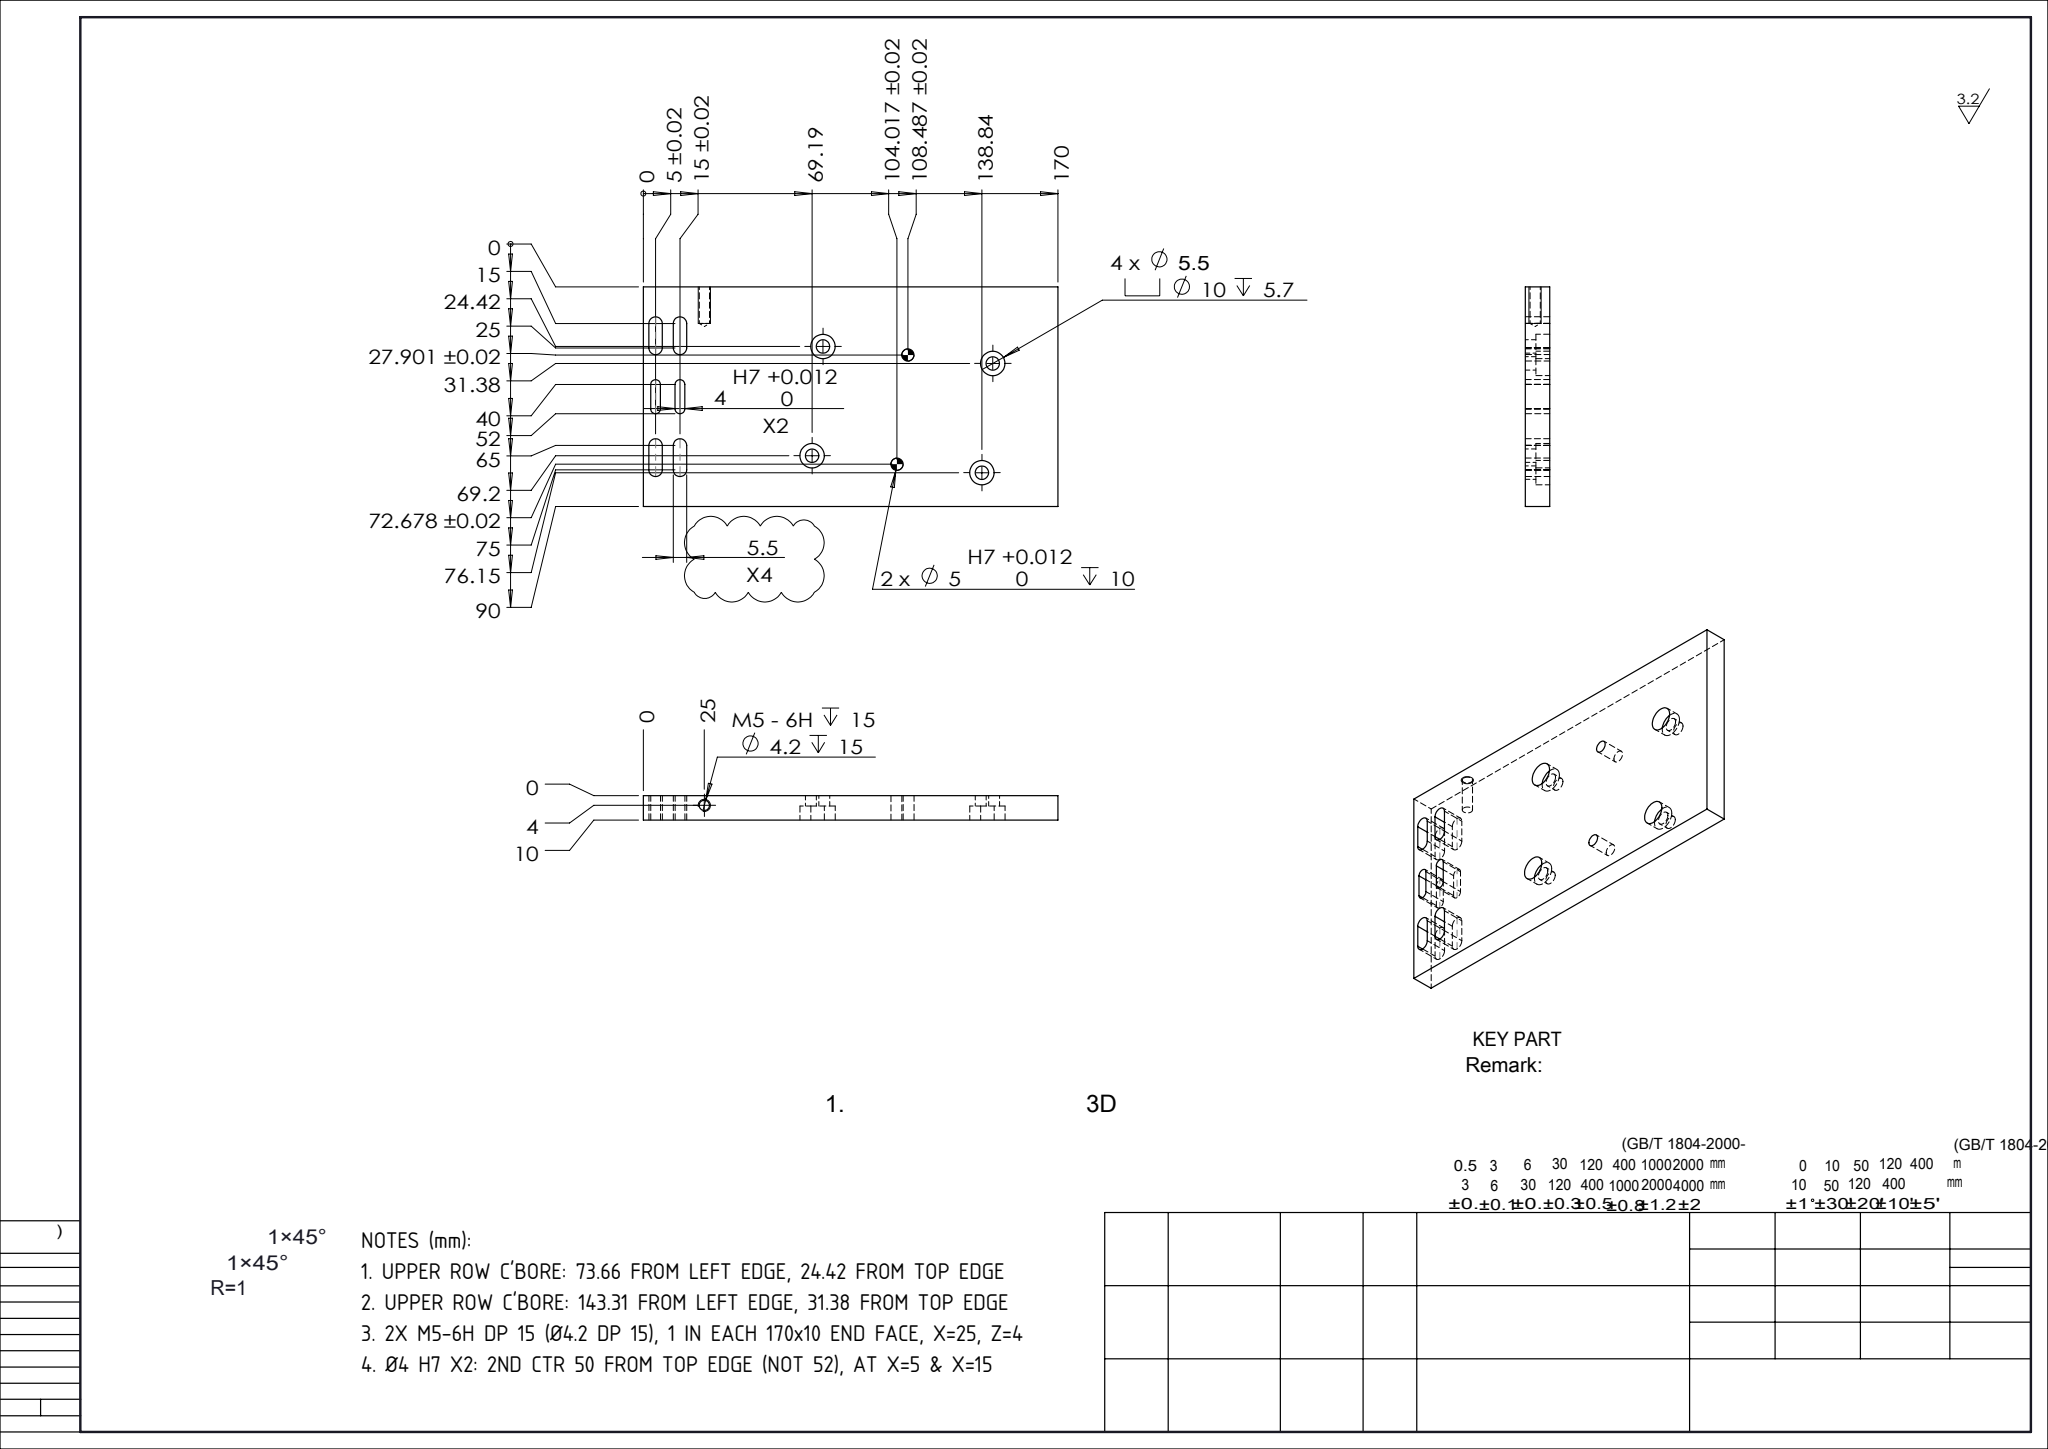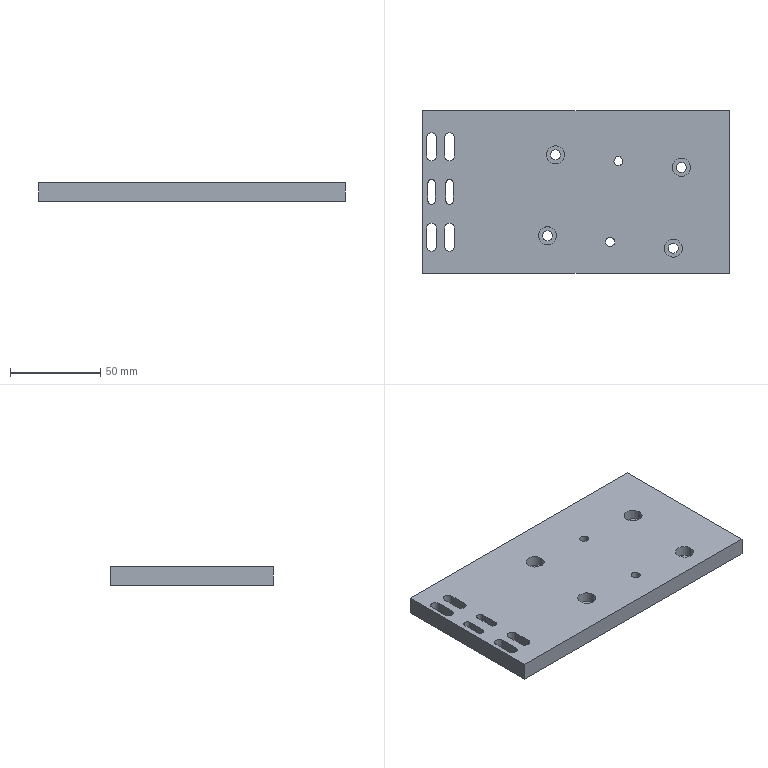Part | SolidWorks | mm | 1 solid | 58 faces | box 170 x 90 x 10 mm | volume 145993 mm3 | cylinder 34 | plane 22 | cone 2 | commonest cylinder face diameters 5.5 x16 10 x8 5 x4 4 x4 4.2 x2
Drawing notes:
UPPER ROW C'BORE: 73.66 FROM LEFT EDGE, 24.42 FROM TOP EDGE | from the solid: Ø5.5 thru w/ Ø10↧5.7 c'bore at x=73.66, y=65.58 (=90-24.42)
UPPER ROW C'BORE: 143.31 FROM LEFT EDGE, 31.38 FROM TOP EDGE | from the solid: Ø5.5 thru w/ Ø10↧5.7 c'bore at x=143.31, y=58.62 (=90-31.38)
2X M5-6H DP 15 (Ø4.2 DP 15), 1 IN EACH 170x10 END FACE, X=25, Z=4 | from the solid: [4.2,'y',[25.0,null,4.0],15.0,2] - two Ø4.2 y-axis holes in y=0 and y=90 faces
Ø4 H7 X2: 2ND CTR 50 FROM TOP EDGE (NOT 52), AT X=5 & X=15 | from the solid: cylinders Ø4 z-axis at [5,50],[15,50] and [5,40],[15,40]; bbox Y=90 so 40 & 50 from top edge
build123d program:
from build123d import *

# Parameters (mm, degrees)
SKETCH1_W                  = 170
SKETCH1_H                  = 90
BOSS_EXTRUDE1_DEPTH        = 10
CUT_EXTRUDE1_DEPTH         = 10
LPATTERN1_COUNT            = 2
LPATTERN1_PITCH            = 50
LPATTERN1_COUNT_DIR2       = 2
LPATTERN1_PITCH_DIR2       = 10
CUT_EXTRUDE2_DEPTH         = 10
HOLE_WIZARD_K_D            = 5.5
HOLE_WIZARD_K_CBORE_D      = 10
HOLE_WIZARD_K_CBORE_DEPTH  = 5.7
SIZE_MM_DOWEL_PIN_HOLE_1_D = 5
M5_TAPPED_HOLE1_D          = 4.2
M5_TAPPED_HOLE1_DEPTH      = 15
M5_TAPPED_HOLE1_TIP        = 1.262


with BuildPart() as part:
    # Sketch1 → Boss-Extrude1 (new body)
    with BuildSketch(Plane.XY):
        Rectangle(SKETCH1_W, SKETCH1_H)
    extrude(amount=BOSS_EXTRUDE1_DEPTH)

    # Sketch2 → Cut-Extrude1 (cut)
    with BuildSketch(Plane(origin=(0, 0, 0), x_dir=(-1, 0, 0), z_dir=(0, 0, -1))):
        with BuildLine():
            Line((82.75, -20), (82.75, -30))
            ThreePointArc((82.75, -30), (80, -32.75), (77.25, -30))
            Line((77.25, -30), (77.25, -20))
            ThreePointArc((77.25, -20), (80, -17.25), (82.75, -20))
        make_face()
    cut_extrude1 = extrude(amount=-CUT_EXTRUDE1_DEPTH, mode=Mode.SUBTRACT)

    # LPattern1: Cut-Extrude1 2 × 2
    with Locations(*[(j * LPATTERN1_PITCH_DIR2, i * LPATTERN1_PITCH, 0) for i in range(LPATTERN1_COUNT) for j in range(LPATTERN1_COUNT_DIR2) if (i, j) != (0, 0)]):
        add(cut_extrude1, mode=Mode.SUBTRACT)

    # Sketch3 → Cut-Extrude2 (cut)
    with BuildSketch(Plane(origin=(0, 0, 0), x_dir=(-1, 0, 0), z_dir=(0, 0, -1))):
        with BuildLine():
            Line((78, -5), (78, 5))
            ThreePointArc((78, 5), (80, 7), (82, 5))
            Line((82, 5), (82, -5))
            ThreePointArc((82, -5), (80, -7), (78, -5))
        make_face()
        with BuildLine():
            Line((68, -5), (68, 5))
            ThreePointArc((68, 5), (70, 7), (72, 5))
            Line((72, 5), (72, -5))
            ThreePointArc((72, -5), (70, -7), (68, -5))
        make_face()
    extrude(amount=-CUT_EXTRUDE2_DEPTH, mode=Mode.SUBTRACT)

    # Hole Wizard K (through all)
    with Locations(Plane.XY.offset(10)):
        with Locations((-11.34, 20.575), (-15.81, -24.202), (58.314, 13.623), (53.844, -31.154)):
            CounterBoreHole(HOLE_WIZARD_K_D / 2, HOLE_WIZARD_K_CBORE_D / 2, HOLE_WIZARD_K_CBORE_DEPTH)

    # Size mm Dowel Pin Hole 1 (through all)
    with Locations(Plane(origin=(0, 0, 0), x_dir=(-1, 0, 0), z_dir=(0, 0, -1))):
        with Locations((-23.487, 17.099), (-19.017, -27.678)):
            Hole(SIZE_MM_DOWEL_PIN_HOLE_1_D / 2)

    # M5 Tapped Hole1
    with Locations(Plane(origin=(0, 45, 0), x_dir=(1, 0, 0), z_dir=(0, 1, 0))):
        with Locations((-60, -4)):
            Hole(M5_TAPPED_HOLE1_D / 2, depth=M5_TAPPED_HOLE1_DEPTH)
            with Locations((0, 0, -(M5_TAPPED_HOLE1_DEPTH + M5_TAPPED_HOLE1_TIP / 2))):  # 118° drill point
                Cone(0, M5_TAPPED_HOLE1_D / 2, M5_TAPPED_HOLE1_TIP, mode=Mode.SUBTRACT)


solid = part.part